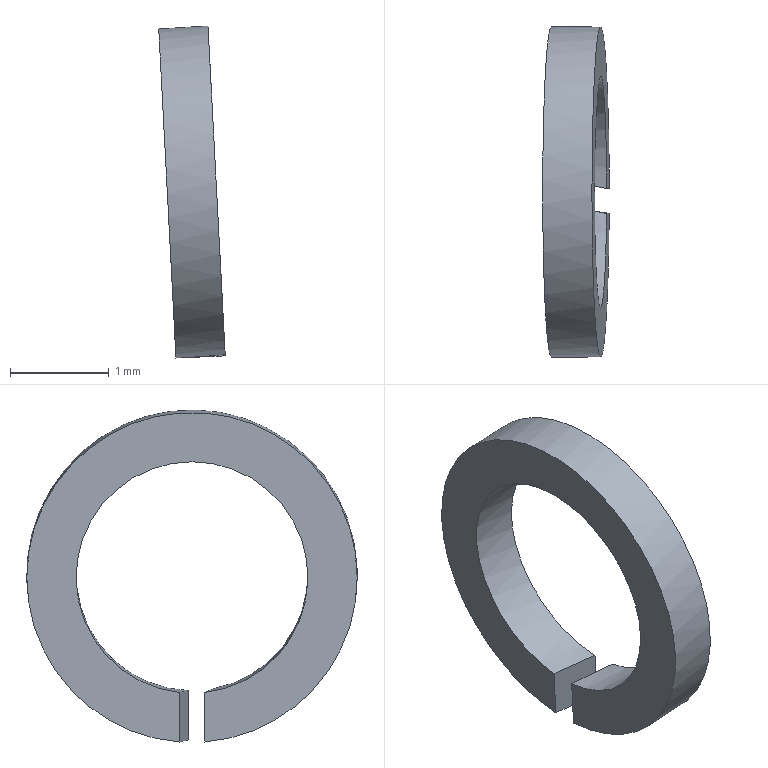Component | NX | GB93-87_2_7 | 1 solid | 6 faces | box 0.67 x 3.35 x 3.37 mm | volume 2 mm3 | plane 4 | cylinder 2 | commonest cylinder face diameters 3.35 x1 2.35 x1
STEP:
#1=CARTESIAN_POINT('',(0.,0.,0.));
#2=DIRECTION('',(0.,0.,1.));
#3=DIRECTION('',(1.,0.,0.));
#4=AXIS2_PLACEMENT_3D('',#1,#2,#3);
#5=CARTESIAN_POINT('',(47.862,-33.952,149.35));
#6=VERTEX_POINT('',#5);
#7=CARTESIAN_POINT('',(47.862,-33.699,149.35));
#8=VERTEX_POINT('',#7);
#9=CARTESIAN_POINT('',(47.775,-33.825,151.018));
#10=DIRECTION('',(-0.9986,0.,-0.05234));
#11=DIRECTION('',(-0.05234,0.,0.9986));
#12=AXIS2_PLACEMENT_3D('',#9,#10,#11);
#13=CIRCLE('',#12,1.675);
#14=CARTESIAN_POINT('',(47.775,-33.825,151.018));
#15=DIRECTION('',(-0.9986,0.,-0.05234));
#16=DIRECTION('',(-0.05234,0.,0.9986));
#17=AXIS2_PLACEMENT_3D('',#14,#15,#16);
#18=CYLINDRICAL_SURFACE('',#17,1.675);
#19=CARTESIAN_POINT('',(-6.283,-0.));
#20=DIRECTION('',(1.,0.));
#21=VECTOR('',#20,1.);
#22=LINE('',#19,#21);
#23=(GEOMETRIC_REPRESENTATION_CONTEXT(2)PARAMETRIC_REPRESENTATION_CONTEXT()REPRESENTATION_CONTEXT('',''));
#24=DEFINITIONAL_REPRESENTATION('',(#22),#23);
#25=PCURVE('',#18,#24);
#26=CARTESIAN_POINT('',(47.775,-32.65,151.018));
#27=DIRECTION('',(-0.9986,0.,-0.05234));
#28=DIRECTION('',(-0.05234,0.,0.9986));
#29=AXIS2_PLACEMENT_3D('',#26,#27,#28);
#30=PLANE('',#29);
#31=CARTESIAN_POINT('',(0.,-1.175));
#32=DIRECTION('',(1.,0.));
#33=AXIS2_PLACEMENT_2D('',#31,#32);
#34=CIRCLE('',#33,1.675);
#35=(GEOMETRIC_REPRESENTATION_CONTEXT(2)PARAMETRIC_REPRESENTATION_CONTEXT()REPRESENTATION_CONTEXT('',''));
#36=DEFINITIONAL_REPRESENTATION('',(#34),#35);
#37=PCURVE('',#30,#36);
#38=SURFACE_CURVE('',#13,(#25,#37),.PCURVE_S1.);
#39=EDGE_CURVE('',#6,#8,#38,.T.);
#40=ORIENTED_EDGE('',*,*,#39,.F.);
#41=CARTESIAN_POINT('',(48.361,-34.041,149.385));
#42=VERTEX_POINT('',#41);
#43=CARTESIAN_POINT('',(47.056,-33.825,150.98));
#44=DIRECTION('',(-0.1734,-0.9848,-0.009088));
#45=DIRECTION('',(-0.9835,0.1736,-0.05154));
#46=AXIS2_PLACEMENT_3D('',#43,#44,#45);
#47=ELLIPSE('',#46,9.646,1.675);
#48=CARTESIAN_POINT('',(-3.066,-0.));
#49=CARTESIAN_POINT('',(-3.013,-0.5));
#50=B_SPLINE_CURVE_WITH_KNOTS('',1,(#48,#49),.UNSPECIFIED.,.F.,.F.,(2,2),(1.647,1.7),.PIECEWISE_BEZIER_KNOTS.);
#51=(GEOMETRIC_REPRESENTATION_CONTEXT(2)PARAMETRIC_REPRESENTATION_CONTEXT()REPRESENTATION_CONTEXT('',''));
#52=DEFINITIONAL_REPRESENTATION('',(#50),#51);
#53=PCURVE('',#18,#52);
#54=CARTESIAN_POINT('',(48.622,-34.079,148.546));
#55=DIRECTION('',(0.1734,0.9848,0.009088));
#56=DIRECTION('',(0.9835,-0.1736,0.05154));
#57=AXIS2_PLACEMENT_3D('',#54,#55,#56);
#58=PLANE('',#57);
#59=CARTESIAN_POINT('',(-11.105,-2.513));
#60=CARTESIAN_POINT('',(-11.105,0.3887));
#61=CARTESIAN_POINT('',(3.364,-1.062));
#62=CARTESIAN_POINT('',(17.833,-2.513));
#63=CARTESIAN_POINT('',(3.364,-3.963));
#64=CARTESIAN_POINT('',(-11.105,-5.414));
#65=CARTESIAN_POINT('',(-11.105,-2.513));
#66=(BOUNDED_CURVE()B_SPLINE_CURVE(2,(#59,#60,#61,#62,#63,#64,#65),.UNSPECIFIED.,.T.,.F.)B_SPLINE_CURVE_WITH_KNOTS((1,2,2,2,2,1),(-2.094,0.,2.094,4.189,6.283,8.378),.UNSPECIFIED.)CURVE()GEOMETRIC_REPRESENTATION_ITEM()RATIONAL_B_SPLINE_CURVE((1.,0.5,1.,0.5,1.,0.5,1.))REPRESENTATION_ITEM(''));
#67=(GEOMETRIC_REPRESENTATION_CONTEXT(2)PARAMETRIC_REPRESENTATION_CONTEXT()REPRESENTATION_CONTEXT('',''));
#68=DEFINITIONAL_REPRESENTATION('',(#66),#67);
#69=PCURVE('',#58,#68);
#70=SURFACE_CURVE('',#47,(#53,#69),.PCURVE_S1.);
#71=EDGE_CURVE('',#6,#42,#70,.T.);
#72=ORIENTED_EDGE('',*,*,#71,.T.);
#73=CARTESIAN_POINT('',(48.362,-33.787,149.372));
#74=VERTEX_POINT('',#73);
#75=CARTESIAN_POINT('',(48.274,-33.825,151.044));
#76=DIRECTION('',(-0.9986,0.,-0.05234));
#77=DIRECTION('',(-0.05234,0.,0.9986));
#78=AXIS2_PLACEMENT_3D('',#75,#76,#77);
#79=CIRCLE('',#78,1.675);
#80=CARTESIAN_POINT('',(-6.283,-0.5));
#81=DIRECTION('',(1.,0.));
#82=VECTOR('',#81,1.);
#83=LINE('',#80,#82);
#84=(GEOMETRIC_REPRESENTATION_CONTEXT(2)PARAMETRIC_REPRESENTATION_CONTEXT()REPRESENTATION_CONTEXT('',''));
#85=DEFINITIONAL_REPRESENTATION('',(#83),#84);
#86=PCURVE('',#18,#85);
#87=CARTESIAN_POINT('',(48.274,-32.15,151.044));
#88=DIRECTION('',(0.9986,0.,0.05234));
#89=DIRECTION('',(0.05234,0.,-0.9986));
#90=AXIS2_PLACEMENT_3D('',#87,#88,#89);
#91=PLANE('',#90);
#92=CARTESIAN_POINT('',(-1.675,-1.675));
#93=CARTESIAN_POINT('',(-1.675,1.226));
#94=CARTESIAN_POINT('',(0.8375,-0.2244));
#95=CARTESIAN_POINT('',(3.35,-1.675));
#96=CARTESIAN_POINT('',(0.8375,-3.126));
#97=CARTESIAN_POINT('',(-1.675,-4.576));
#98=CARTESIAN_POINT('',(-1.675,-1.675));
#99=(BOUNDED_CURVE()B_SPLINE_CURVE(2,(#92,#93,#94,#95,#96,#97,#98),.UNSPECIFIED.,.T.,.F.)B_SPLINE_CURVE_WITH_KNOTS((1,2,2,2,2,1),(-2.094,0.,2.094,4.189,6.283,8.378),.UNSPECIFIED.)CURVE()GEOMETRIC_REPRESENTATION_ITEM()RATIONAL_B_SPLINE_CURVE((1.,0.5,1.,0.5,1.,0.5,1.))REPRESENTATION_ITEM(''));
#100=(GEOMETRIC_REPRESENTATION_CONTEXT(2)PARAMETRIC_REPRESENTATION_CONTEXT()REPRESENTATION_CONTEXT('',''));
#101=DEFINITIONAL_REPRESENTATION('',(#99),#100);
#102=PCURVE('',#91,#101);
#103=SURFACE_CURVE('',#79,(#86,#102),.PCURVE_S1.);
#104=EDGE_CURVE('',#42,#74,#103,.T.);
#105=ORIENTED_EDGE('',*,*,#104,.T.);
#106=CARTESIAN_POINT('',(48.493,-33.825,151.056));
#107=DIRECTION('',(0.1734,0.9848,0.009088));
#108=DIRECTION('',(-0.9835,0.1736,-0.05154));
#109=AXIS2_PLACEMENT_3D('',#106,#107,#108);
#110=ELLIPSE('',#109,9.646,1.675);
#111=CARTESIAN_POINT('',(3.118,-0.5));
#112=CARTESIAN_POINT('',(3.066,-0.));
#113=B_SPLINE_CURVE_WITH_KNOTS('',1,(#111,#112),.UNSPECIFIED.,.F.,.F.,(2,2),(4.736,4.788),.PIECEWISE_BEZIER_KNOTS.);
#114=(GEOMETRIC_REPRESENTATION_CONTEXT(2)PARAMETRIC_REPRESENTATION_CONTEXT()REPRESENTATION_CONTEXT('',''));
#115=DEFINITIONAL_REPRESENTATION('',(#113),#114);
#116=PCURVE('',#18,#115);
#117=CARTESIAN_POINT('',(47.19,-33.572,148.471));
#118=DIRECTION('',(-0.1734,-0.9848,-0.009088));
#119=DIRECTION('',(-0.9835,0.1736,-0.05154));
#120=AXIS2_PLACEMENT_3D('',#117,#118,#119);
#121=PLANE('',#120);
#122=CARTESIAN_POINT('',(8.187,-2.513));
#123=CARTESIAN_POINT('',(8.187,-5.414));
#124=CARTESIAN_POINT('',(-6.282,-3.963));
#125=CARTESIAN_POINT('',(-20.751,-2.513));
#126=CARTESIAN_POINT('',(-6.282,-1.062));
#127=CARTESIAN_POINT('',(8.187,0.3887));
#128=CARTESIAN_POINT('',(8.187,-2.513));
#129=(BOUNDED_CURVE()B_SPLINE_CURVE(2,(#122,#123,#124,#125,#126,#127,#128),.UNSPECIFIED.,.T.,.F.)B_SPLINE_CURVE_WITH_KNOTS((1,2,2,2,2,1),(-2.094,0.,2.094,4.189,6.283,8.378),.UNSPECIFIED.)CURVE()GEOMETRIC_REPRESENTATION_ITEM()RATIONAL_B_SPLINE_CURVE((1.,0.5,1.,0.5,1.,0.5,1.))REPRESENTATION_ITEM(''));
#130=(GEOMETRIC_REPRESENTATION_CONTEXT(2)PARAMETRIC_REPRESENTATION_CONTEXT()REPRESENTATION_CONTEXT('',''));
#131=DEFINITIONAL_REPRESENTATION('',(#129),#130);
#132=PCURVE('',#121,#131);
#133=SURFACE_CURVE('',#110,(#116,#132),.PCURVE_S1.);
#134=EDGE_CURVE('',#74,#8,#133,.T.);
#135=ORIENTED_EDGE('',*,*,#134,.T.);
#136=EDGE_LOOP('',(#40,#72,#105,#135));
#137=FACE_BOUND('',#136,.T.);
#138=ADVANCED_FACE('',(#137),#18,.T.);
#139=ORIENTED_EDGE('',*,*,#104,.F.);
#140=CARTESIAN_POINT('',(48.334,-34.041,149.891));
#141=VERTEX_POINT('',#140);
#142=CARTESIAN_POINT('',(48.274,-34.041,151.044));
#143=DIRECTION('',(-0.05234,0.,0.9986));
#144=VECTOR('',#143,1.);
#145=LINE('',#142,#144);
#146=CARTESIAN_POINT('',(0.,-1.89));
#147=DIRECTION('',(-1.,0.));
#148=VECTOR('',#147,1.);
#149=LINE('',#146,#148);
#150=(GEOMETRIC_REPRESENTATION_CONTEXT(2)PARAMETRIC_REPRESENTATION_CONTEXT()REPRESENTATION_CONTEXT('',''));
#151=DEFINITIONAL_REPRESENTATION('',(#149),#150);
#152=PCURVE('',#91,#151);
#153=CARTESIAN_POINT('',(-0.2202,-2.513));
#154=DIRECTION('',(-0.,-1.));
#155=VECTOR('',#154,1.);
#156=LINE('',#153,#155);
#157=(GEOMETRIC_REPRESENTATION_CONTEXT(2)PARAMETRIC_REPRESENTATION_CONTEXT()REPRESENTATION_CONTEXT('',''));
#158=DEFINITIONAL_REPRESENTATION('',(#156),#157);
#159=PCURVE('',#58,#158);
#160=SURFACE_CURVE('',#145,(#152,#159),.PCURVE_S1.);
#161=EDGE_CURVE('',#42,#141,#160,.T.);
#162=ORIENTED_EDGE('',*,*,#161,.T.);
#163=CARTESIAN_POINT('',(48.335,-33.787,149.871));
#164=VERTEX_POINT('',#163);
#165=CARTESIAN_POINT('',(48.274,-33.825,151.044));
#166=DIRECTION('',(-0.9986,0.,-0.05234));
#167=DIRECTION('',(-0.05234,0.,0.9986));
#168=AXIS2_PLACEMENT_3D('',#165,#166,#167);
#169=CIRCLE('',#168,1.175);
#170=CARTESIAN_POINT('',(-1.175,-1.675));
#171=CARTESIAN_POINT('',(-1.175,0.3602));
#172=CARTESIAN_POINT('',(0.5875,-0.6574));
#173=CARTESIAN_POINT('',(2.35,-1.675));
#174=CARTESIAN_POINT('',(0.5875,-2.693));
#175=CARTESIAN_POINT('',(-1.175,-3.71));
#176=CARTESIAN_POINT('',(-1.175,-1.675));
#177=(BOUNDED_CURVE()B_SPLINE_CURVE(2,(#170,#171,#172,#173,#174,#175,#176),.UNSPECIFIED.,.T.,.F.)B_SPLINE_CURVE_WITH_KNOTS((1,2,2,2,2,1),(-2.094,0.,2.094,4.189,6.283,8.378),.UNSPECIFIED.)CURVE()GEOMETRIC_REPRESENTATION_ITEM()RATIONAL_B_SPLINE_CURVE((1.,0.5,1.,0.5,1.,0.5,1.))REPRESENTATION_ITEM(''));
#178=(GEOMETRIC_REPRESENTATION_CONTEXT(2)PARAMETRIC_REPRESENTATION_CONTEXT()REPRESENTATION_CONTEXT('',''));
#179=DEFINITIONAL_REPRESENTATION('',(#177),#178);
#180=PCURVE('',#91,#179);
#181=CARTESIAN_POINT('',(47.775,-33.825,151.018));
#182=DIRECTION('',(-0.9986,0.,-0.05234));
#183=DIRECTION('',(-0.05234,0.,0.9986));
#184=AXIS2_PLACEMENT_3D('',#181,#182,#183);
#185=CYLINDRICAL_SURFACE('',#184,1.175);
#186=CARTESIAN_POINT('',(-6.283,-0.5));
#187=DIRECTION('',(1.,0.));
#188=VECTOR('',#187,1.);
#189=LINE('',#186,#188);
#190=(GEOMETRIC_REPRESENTATION_CONTEXT(2)PARAMETRIC_REPRESENTATION_CONTEXT()REPRESENTATION_CONTEXT('',''));
#191=DEFINITIONAL_REPRESENTATION('',(#189),#190);
#192=PCURVE('',#185,#191);
#193=SURFACE_CURVE('',#169,(#180,#192),.PCURVE_S1.);
#194=EDGE_CURVE('',#141,#164,#193,.T.);
#195=ORIENTED_EDGE('',*,*,#194,.T.);
#196=CARTESIAN_POINT('',(48.274,-33.787,151.044));
#197=DIRECTION('',(0.05234,0.,-0.9986));
#198=VECTOR('',#197,1.);
#199=LINE('',#196,#198);
#200=CARTESIAN_POINT('',(0.,-1.636));
#201=DIRECTION('',(1.,0.));
#202=VECTOR('',#201,1.);
#203=LINE('',#200,#202);
#204=(GEOMETRIC_REPRESENTATION_CONTEXT(2)PARAMETRIC_REPRESENTATION_CONTEXT()REPRESENTATION_CONTEXT('',''));
#205=DEFINITIONAL_REPRESENTATION('',(#203),#204);
#206=PCURVE('',#91,#205);
#207=CARTESIAN_POINT('',(-1.236,-2.513));
#208=DIRECTION('',(-0.,1.));
#209=VECTOR('',#208,1.);
#210=LINE('',#207,#209);
#211=(GEOMETRIC_REPRESENTATION_CONTEXT(2)PARAMETRIC_REPRESENTATION_CONTEXT()REPRESENTATION_CONTEXT('',''));
#212=DEFINITIONAL_REPRESENTATION('',(#210),#211);
#213=PCURVE('',#121,#212);
#214=SURFACE_CURVE('',#199,(#206,#213),.PCURVE_S1.);
#215=EDGE_CURVE('',#164,#74,#214,.T.);
#216=ORIENTED_EDGE('',*,*,#215,.T.);
#217=EDGE_LOOP('',(#139,#162,#195,#216));
#218=FACE_BOUND('',#217,.T.);
#219=ADVANCED_FACE('',(#218),#91,.T.);
#220=CARTESIAN_POINT('',(47.836,-33.699,149.851));
#221=VERTEX_POINT('',#220);
#222=CARTESIAN_POINT('',(48.493,-33.825,151.056));
#223=DIRECTION('',(-0.1734,-0.9848,-0.009088));
#224=DIRECTION('',(-0.9835,0.1736,-0.05154));
#225=AXIS2_PLACEMENT_3D('',#222,#223,#224);
#226=ELLIPSE('',#225,6.767,1.175);
#227=CARTESIAN_POINT('',(3.033,-0.));
#228=CARTESIAN_POINT('',(3.109,-0.5));
#229=B_SPLINE_CURVE_WITH_KNOTS('',1,(#227,#228),.UNSPECIFIED.,.F.,.F.,(2,2),(1.463,1.538),.PIECEWISE_BEZIER_KNOTS.);
#230=(GEOMETRIC_REPRESENTATION_CONTEXT(2)PARAMETRIC_REPRESENTATION_CONTEXT()REPRESENTATION_CONTEXT('',''));
#231=DEFINITIONAL_REPRESENTATION('',(#229),#230);
#232=PCURVE('',#185,#231);
#233=CARTESIAN_POINT('',(-1.459,-2.513));
#234=DIRECTION('',(1.,0.));
#235=AXIS2_PLACEMENT_2D('',#233,#234);
#236=ELLIPSE('',#235,6.767,1.175);
#237=(GEOMETRIC_REPRESENTATION_CONTEXT(2)PARAMETRIC_REPRESENTATION_CONTEXT()REPRESENTATION_CONTEXT('',''));
#238=DEFINITIONAL_REPRESENTATION('',(#236),#237);
#239=PCURVE('',#121,#238);
#240=SURFACE_CURVE('',#226,(#232,#239),.PCURVE_S1.);
#241=EDGE_CURVE('',#221,#164,#240,.T.);
#242=ORIENTED_EDGE('',*,*,#241,.F.);
#243=CARTESIAN_POINT('',(47.836,-33.952,149.851));
#244=VERTEX_POINT('',#243);
#245=CARTESIAN_POINT('',(47.775,-33.825,151.018));
#246=DIRECTION('',(-0.9986,0.,-0.05234));
#247=DIRECTION('',(-0.05234,0.,0.9986));
#248=AXIS2_PLACEMENT_3D('',#245,#246,#247);
#249=CIRCLE('',#248,1.175);
#250=CARTESIAN_POINT('',(-6.283,0.));
#251=DIRECTION('',(1.,0.));
#252=VECTOR('',#251,1.);
#253=LINE('',#250,#252);
#254=(GEOMETRIC_REPRESENTATION_CONTEXT(2)PARAMETRIC_REPRESENTATION_CONTEXT()REPRESENTATION_CONTEXT('',''));
#255=DEFINITIONAL_REPRESENTATION('',(#253),#254);
#256=PCURVE('',#185,#255);
#257=CARTESIAN_POINT('',(0.,-1.175));
#258=DIRECTION('',(1.,0.));
#259=AXIS2_PLACEMENT_2D('',#257,#258);
#260=CIRCLE('',#259,1.175);
#261=(GEOMETRIC_REPRESENTATION_CONTEXT(2)PARAMETRIC_REPRESENTATION_CONTEXT()REPRESENTATION_CONTEXT('',''));
#262=DEFINITIONAL_REPRESENTATION('',(#260),#261);
#263=PCURVE('',#30,#262);
#264=SURFACE_CURVE('',#249,(#256,#263),.PCURVE_S1.);
#265=EDGE_CURVE('',#244,#221,#264,.T.);
#266=ORIENTED_EDGE('',*,*,#265,.F.);
#267=CARTESIAN_POINT('',(47.056,-33.825,150.98));
#268=DIRECTION('',(0.1734,0.9848,0.009088));
#269=DIRECTION('',(-0.9835,0.1736,-0.05154));
#270=AXIS2_PLACEMENT_3D('',#267,#268,#269);
#271=ELLIPSE('',#270,6.767,1.175);
#272=CARTESIAN_POINT('',(-2.957,-0.5));
#273=CARTESIAN_POINT('',(-3.033,-0.));
#274=B_SPLINE_CURVE_WITH_KNOTS('',1,(#272,#273),.UNSPECIFIED.,.F.,.F.,(2,2),(4.528,4.604),.PIECEWISE_BEZIER_KNOTS.);
#275=(GEOMETRIC_REPRESENTATION_CONTEXT(2)PARAMETRIC_REPRESENTATION_CONTEXT()REPRESENTATION_CONTEXT('',''));
#276=DEFINITIONAL_REPRESENTATION('',(#274),#275);
#277=PCURVE('',#185,#276);
#278=CARTESIAN_POINT('',(-1.459,-2.513));
#279=DIRECTION('',(-1.,0.));
#280=AXIS2_PLACEMENT_2D('',#278,#279);
#281=ELLIPSE('',#280,6.767,1.175);
#282=(GEOMETRIC_REPRESENTATION_CONTEXT(2)PARAMETRIC_REPRESENTATION_CONTEXT()REPRESENTATION_CONTEXT('',''));
#283=DEFINITIONAL_REPRESENTATION('',(#281),#282);
#284=PCURVE('',#58,#283);
#285=SURFACE_CURVE('',#271,(#277,#284),.PCURVE_S1.);
#286=EDGE_CURVE('',#141,#244,#285,.T.);
#287=ORIENTED_EDGE('',*,*,#286,.F.);
#288=ORIENTED_EDGE('',*,*,#194,.T.);
#289=EDGE_LOOP('',(#242,#266,#287,#288));
#290=FACE_BOUND('',#289,.F.);
#291=ADVANCED_FACE('',(#290),#185,.F.);
#292=ORIENTED_EDGE('',*,*,#265,.F.);
#293=CARTESIAN_POINT('',(47.775,-33.952,151.018));
#294=DIRECTION('',(0.05234,0.,-0.9986));
#295=VECTOR('',#294,1.);
#296=LINE('',#293,#295);
#297=CARTESIAN_POINT('',(0.,-1.302));
#298=DIRECTION('',(-1.,0.));
#299=VECTOR('',#298,1.);
#300=LINE('',#297,#299);
#301=(GEOMETRIC_REPRESENTATION_CONTEXT(2)PARAMETRIC_REPRESENTATION_CONTEXT()REPRESENTATION_CONTEXT('',''));
#302=DEFINITIONAL_REPRESENTATION('',(#300),#301);
#303=PCURVE('',#30,#302);
#304=CARTESIAN_POINT('',(-0.728,-2.513));
#305=DIRECTION('',(0.,1.));
#306=VECTOR('',#305,1.);
#307=LINE('',#304,#306);
#308=(GEOMETRIC_REPRESENTATION_CONTEXT(2)PARAMETRIC_REPRESENTATION_CONTEXT()REPRESENTATION_CONTEXT('',''));
#309=DEFINITIONAL_REPRESENTATION('',(#307),#308);
#310=PCURVE('',#58,#309);
#311=SURFACE_CURVE('',#296,(#303,#310),.PCURVE_S1.);
#312=EDGE_CURVE('',#244,#6,#311,.T.);
#313=ORIENTED_EDGE('',*,*,#312,.T.);
#314=ORIENTED_EDGE('',*,*,#39,.T.);
#315=CARTESIAN_POINT('',(47.775,-33.699,151.018));
#316=DIRECTION('',(-0.05234,0.,0.9986));
#317=VECTOR('',#316,1.);
#318=LINE('',#315,#317);
#319=CARTESIAN_POINT('',(0.,-1.048));
#320=DIRECTION('',(1.,0.));
#321=VECTOR('',#320,1.);
#322=LINE('',#319,#321);
#323=(GEOMETRIC_REPRESENTATION_CONTEXT(2)PARAMETRIC_REPRESENTATION_CONTEXT()REPRESENTATION_CONTEXT('',''));
#324=DEFINITIONAL_REPRESENTATION('',(#322),#323);
#325=PCURVE('',#30,#324);
#326=CARTESIAN_POINT('',(-0.728,-2.513));
#327=DIRECTION('',(0.,-1.));
#328=VECTOR('',#327,1.);
#329=LINE('',#326,#328);
#330=(GEOMETRIC_REPRESENTATION_CONTEXT(2)PARAMETRIC_REPRESENTATION_CONTEXT()REPRESENTATION_CONTEXT('',''));
#331=DEFINITIONAL_REPRESENTATION('',(#329),#330);
#332=PCURVE('',#121,#331);
#333=SURFACE_CURVE('',#318,(#325,#332),.PCURVE_S1.);
#334=EDGE_CURVE('',#8,#221,#333,.T.);
#335=ORIENTED_EDGE('',*,*,#334,.T.);
#336=EDGE_LOOP('',(#292,#313,#314,#335));
#337=FACE_BOUND('',#336,.T.);
#338=ADVANCED_FACE('',(#337),#30,.T.);
#339=ORIENTED_EDGE('',*,*,#215,.F.);
#340=ORIENTED_EDGE('',*,*,#241,.F.);
#341=ORIENTED_EDGE('',*,*,#334,.F.);
#342=ORIENTED_EDGE('',*,*,#134,.F.);
#343=EDGE_LOOP('',(#339,#340,#341,#342));
#344=FACE_BOUND('',#343,.T.);
#345=ADVANCED_FACE('',(#344),#121,.T.);
#346=ORIENTED_EDGE('',*,*,#312,.F.);
#347=ORIENTED_EDGE('',*,*,#286,.F.);
#348=ORIENTED_EDGE('',*,*,#161,.F.);
#349=ORIENTED_EDGE('',*,*,#71,.F.);
#350=EDGE_LOOP('',(#346,#347,#348,#349));
#351=FACE_BOUND('',#350,.T.);
#352=ADVANCED_FACE('',(#351),#58,.T.);
#353=CLOSED_SHELL('',(#138,#219,#291,#338,#345,#352));
#354=MANIFOLD_SOLID_BREP('',#353);
#355=(LENGTH_UNIT()NAMED_UNIT(*)SI_UNIT(.MILLI.,.METRE.));
#356=UNCERTAINTY_MEASURE_WITH_UNIT(LENGTH_MEASURE(0.0002),#355,'','');
#357=(NAMED_UNIT(*)PLANE_ANGLE_UNIT()SI_UNIT($,.RADIAN.));
#358=(NAMED_UNIT(*)SI_UNIT($,.STERADIAN.)SOLID_ANGLE_UNIT());
#359=(GEOMETRIC_REPRESENTATION_CONTEXT(3)GLOBAL_UNCERTAINTY_ASSIGNED_CONTEXT((#356))GLOBAL_UNIT_ASSIGNED_CONTEXT((#355,#357,#358))REPRESENTATION_CONTEXT('',''));
#360=ADVANCED_BREP_SHAPE_REPRESENTATION('',(#4,#354),#359);